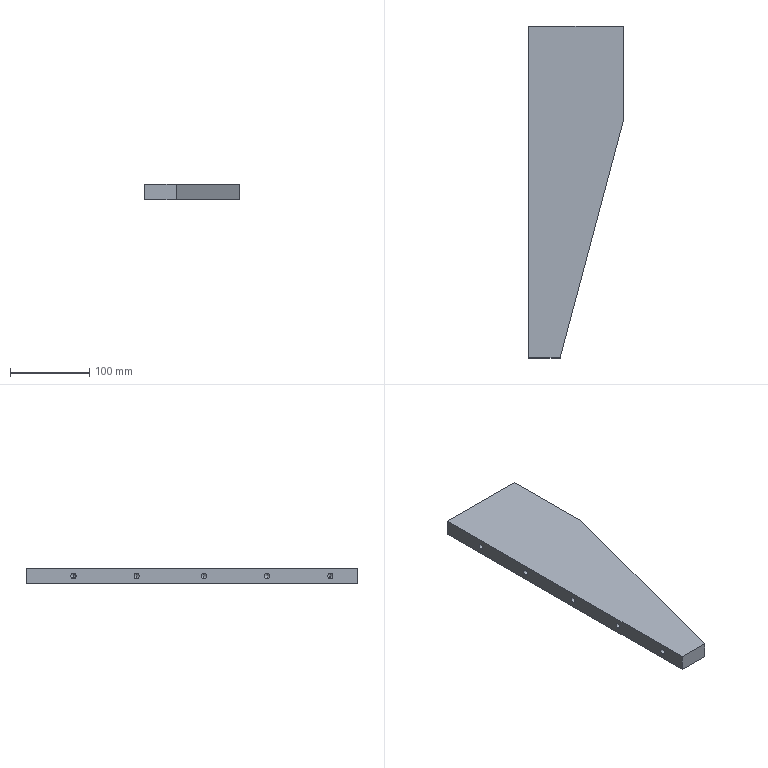Component | SolidWorks | F3-2 | 1 solid | 39 faces | box 120 x 420 x 20 mm | volume 762064 mm3 | cylinder 16 | cone 16 | plane 7 | commonest cylinder face diameters 6.8 x16
build123d program:
from build123d import *

# Parameters (mm, degrees)
BOSS_EXTRUDE1_DEPTH   = 20
M8_TAPPED_HOLE1_D     = 6.8
M8_TAPPED_HOLE1_DEPTH = 19.75
M8_TAPPED_HOLE1_TIP   = 2.043
M8_TAPPED_HOLE2_D     = 6.8
M8_TAPPED_HOLE2_DEPTH = 19.75
M8_TAPPED_HOLE2_TIP   = 2.043


with BuildPart() as part:
    # Sketch1 → Boss-Extrude1 (new body)
    with BuildSketch(Plane.XY):
        Polygon((-112.974, 3095.561), (-112.974, 3515.561), (-232.974, 3515.561), (-232.974, 3395.561), (-152.974, 3095.561), align=None)
    extrude(amount=BOSS_EXTRUDE1_DEPTH)

    # M8 Tapped Hole1
    with Locations(Plane(origin=(0, 3515.561, 0), x_dir=(-1, 0, 0), z_dir=(0, 1, 0))):
        with Locations((130.474, 10), (172.974, 10), (215.474, 10)):
            Hole(M8_TAPPED_HOLE1_D / 2, depth=M8_TAPPED_HOLE1_DEPTH)
            with Locations((0, 0, -(M8_TAPPED_HOLE1_DEPTH + M8_TAPPED_HOLE1_TIP / 2))):  # 118° drill point
                Cone(0, M8_TAPPED_HOLE1_D / 2, M8_TAPPED_HOLE1_TIP, mode=Mode.SUBTRACT)

    # M8 Tapped Hole2
    with Locations(Plane(origin=(-112.974, 0, 0), x_dir=(0, 0, -1), z_dir=(1, 0, 0))):
        with Locations((-10, 3130.561), (-10, 3210.561), (-10, 3375.561), (-10, 3455.561), (-10, 3290.561)):
            Hole(M8_TAPPED_HOLE2_D / 2, depth=M8_TAPPED_HOLE2_DEPTH)
            with Locations((0, 0, -(M8_TAPPED_HOLE2_DEPTH + M8_TAPPED_HOLE2_TIP / 2))):  # 118° drill point
                Cone(0, M8_TAPPED_HOLE2_D / 2, M8_TAPPED_HOLE2_TIP, mode=Mode.SUBTRACT)


solid = part.part

# Placed as in the assembly
solid = solid.moved(Location((8.026, -2923.282, 25), (-180, 0, 180)))